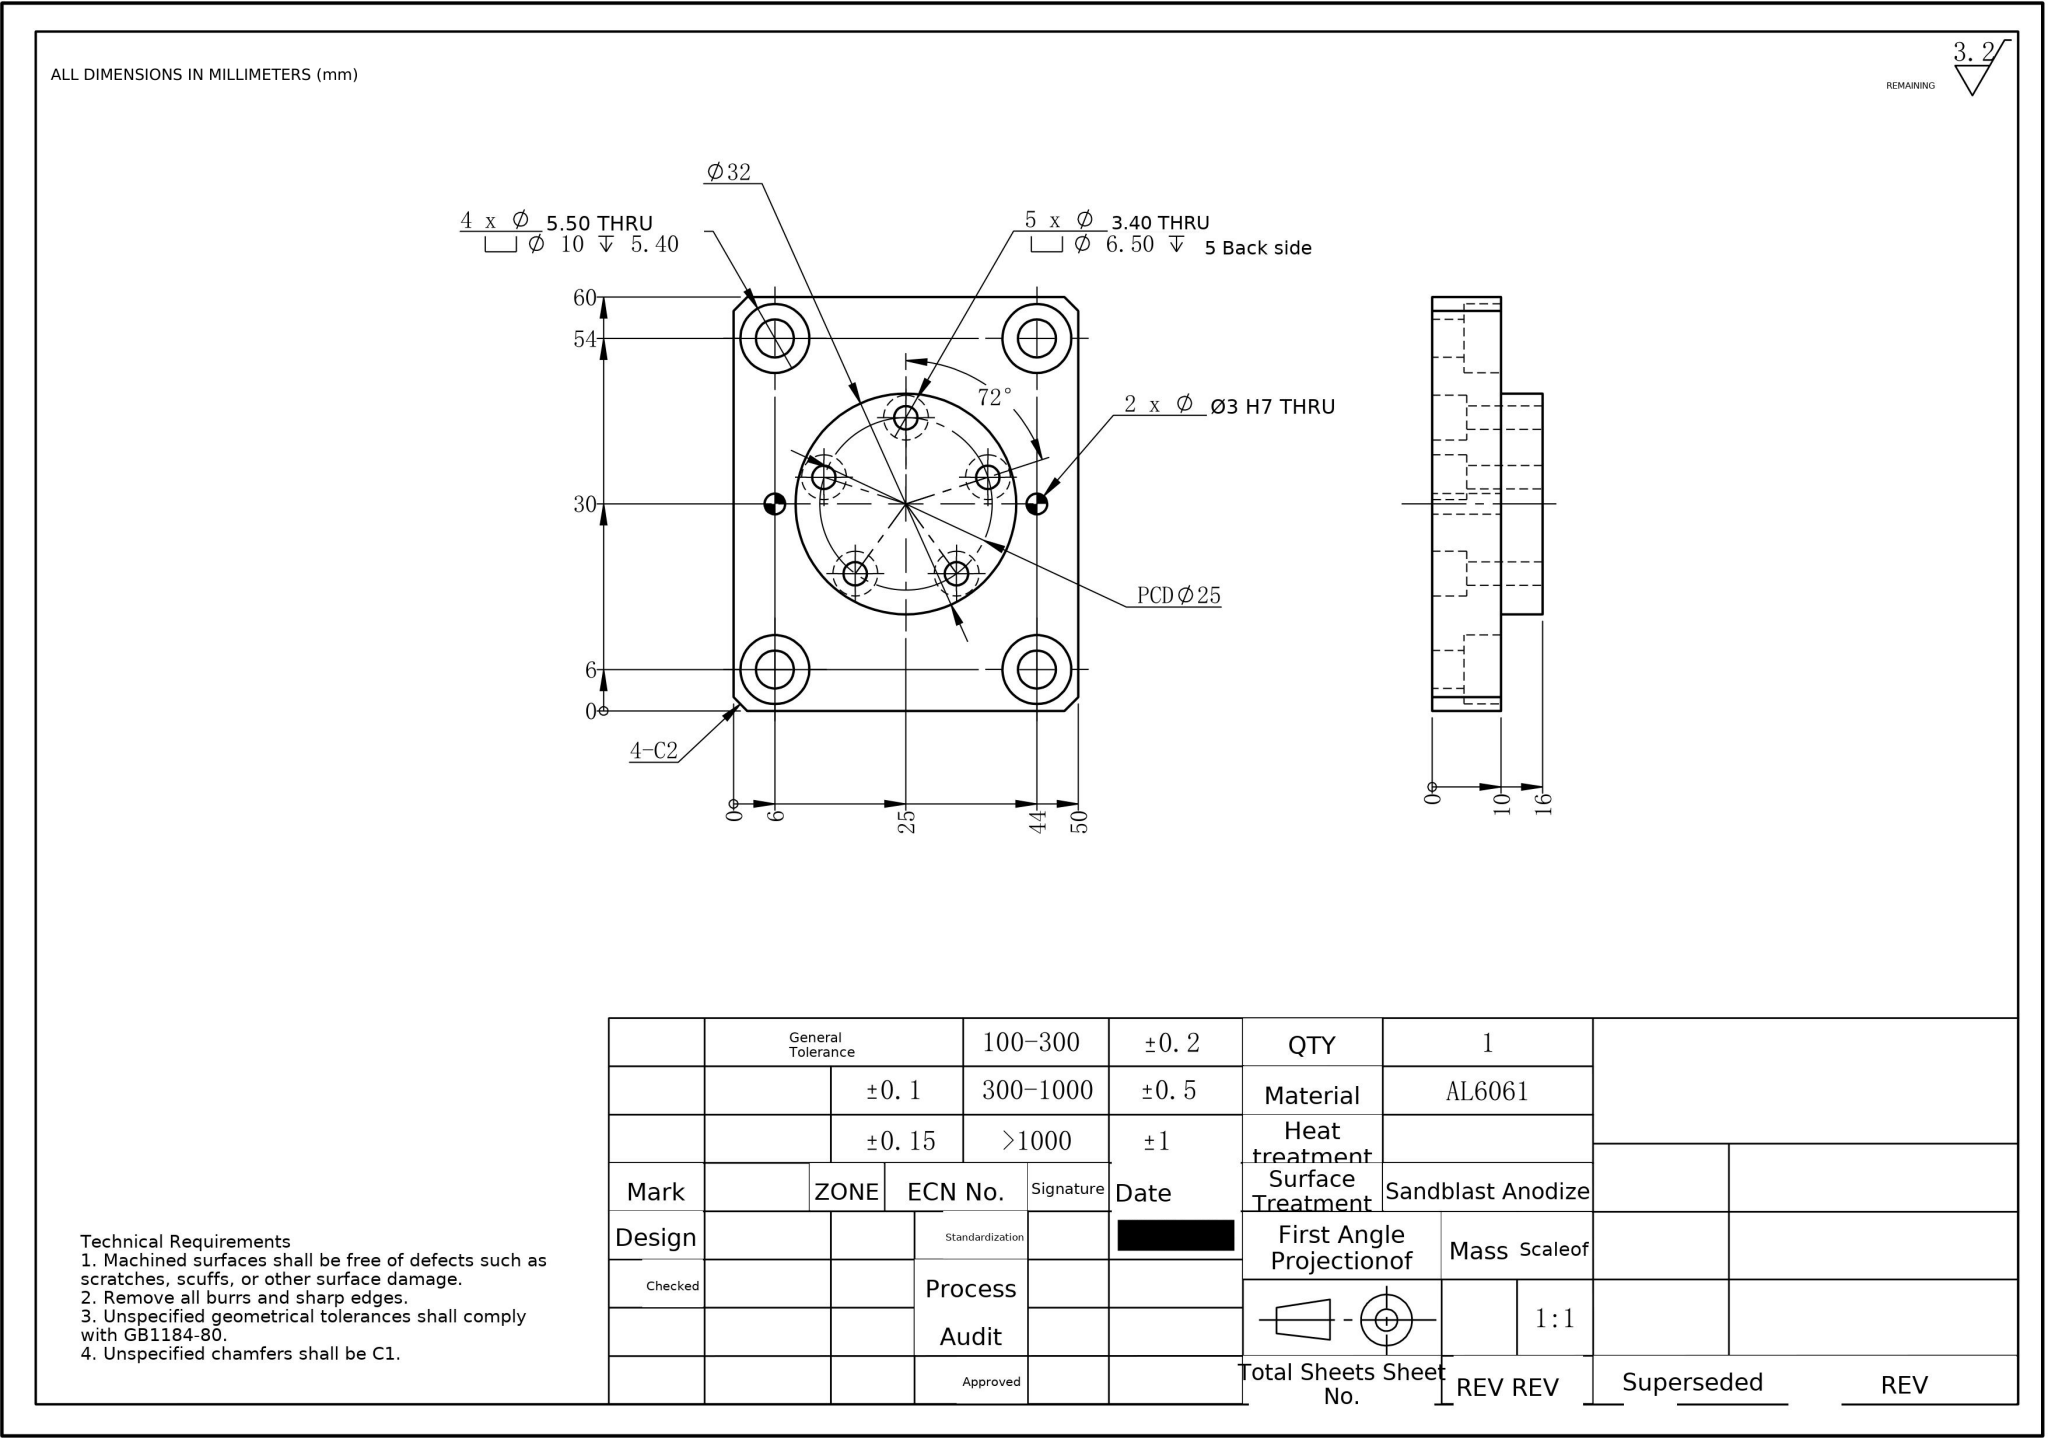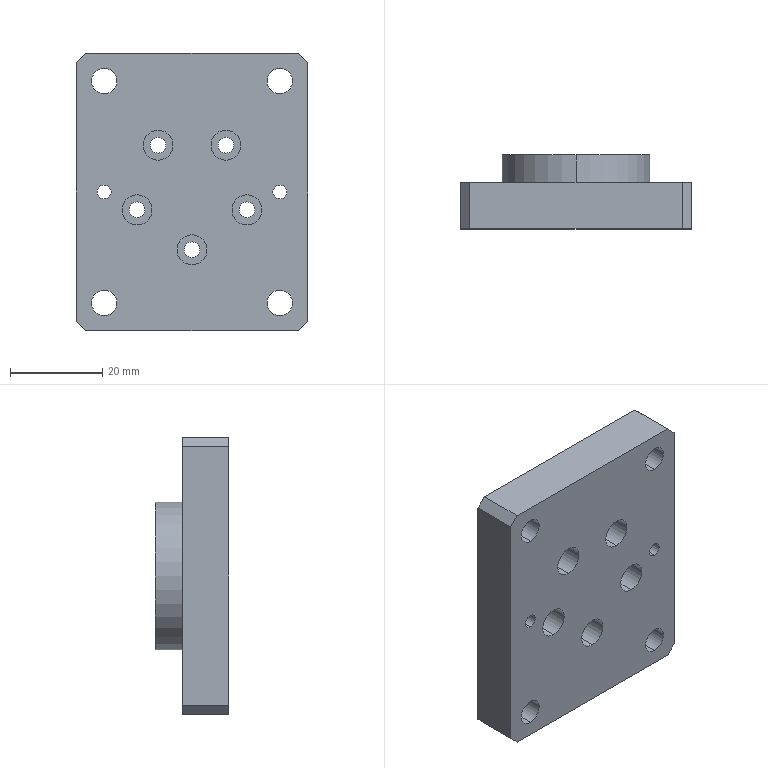Part | NX | mm | 1 solid | 62 faces | box 50 x 16 x 60 mm | volume 31142 mm3 | cylinder 42 | plane 20 | commonest cylinder face diameters 6.5 x10 3.4 x10 10 x8 5.5 x8 3 x4 32 x2